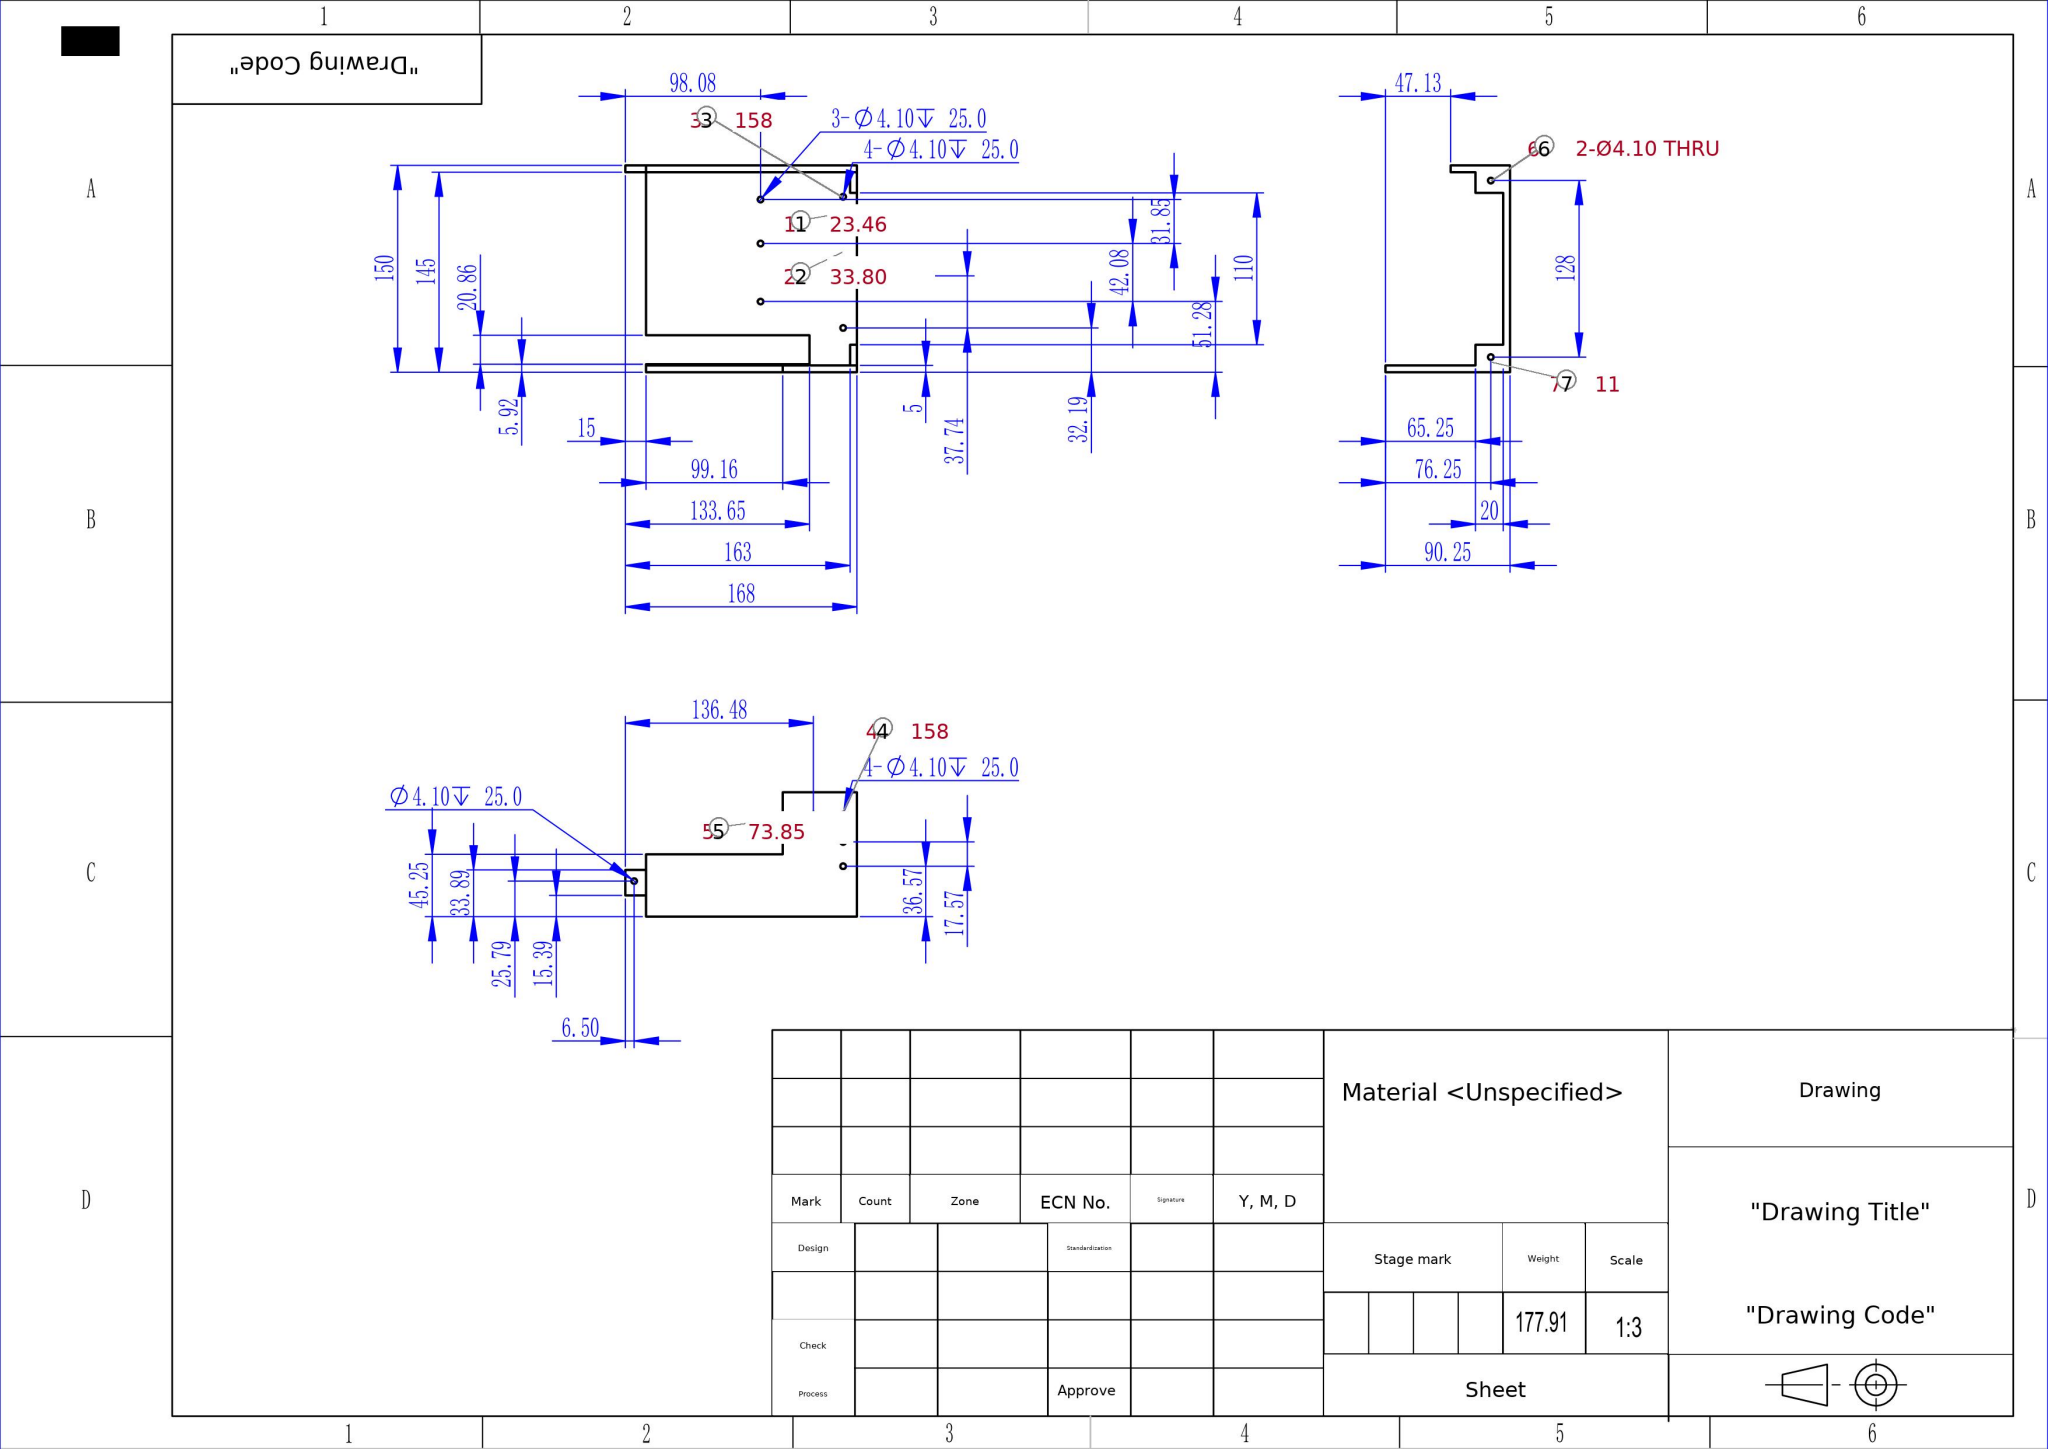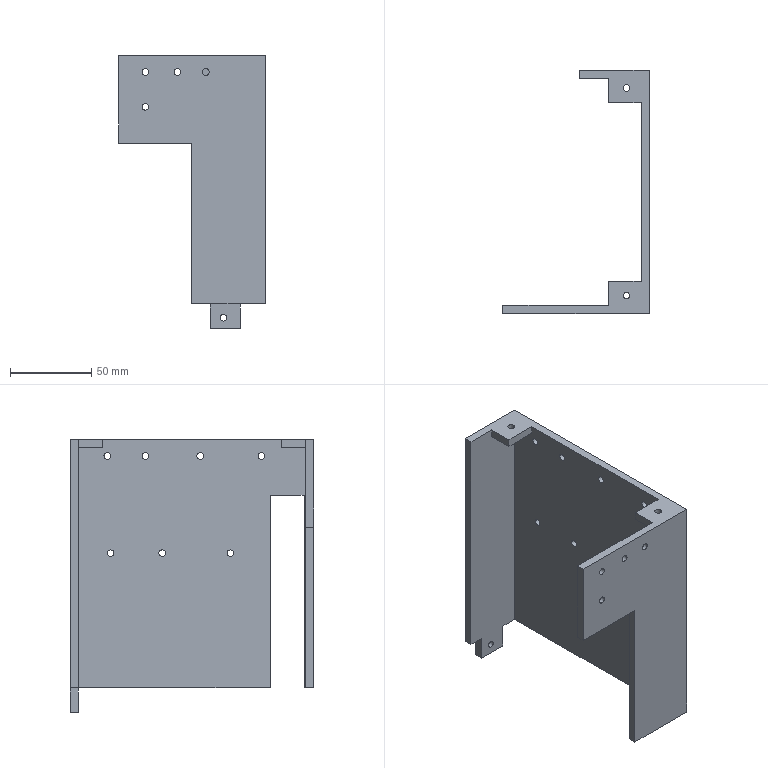Part | SolidWorks | mm | material Unspecified | 1 solid | 54 faces | box 90.25 x 150 x 168 mm | volume 177906 mm3 | cylinder 28 | plane 26 | commonest cylinder face diameters 4.1 x28
build123d program:
from build123d import *

# Parameters (mm, degrees)
BOSS_EXTRUDE1_DEPTH = 153
SKETCH2_W           = 45
SKETCH2_H           = 103.788
CUT_EXTRUDE2_DEPTH  = 104
SKETCH3_W           = 124.99
SKETCH3_H           = 20.86
CUT_EXTRUDE3_DEPTH  = 57
SKETCH4_W           = 20
SKETCH4_H           = 15
SKETCH4_R           = 2.05
BOSS_EXTRUDE2_DEPTH = 5
SKETCH5_W           = 18.5
SKETCH5_H           = 5
BOSS_EXTRUDE3_DEPTH = 15
SKETCH6_R           = 2.05
CUT_EXTRUDE4_DEPTH  = 25
SKETCH7_R           = 2.05
CUT_EXTRUDE5_DEPTH  = 25
SKETCH8_R           = 2.05
CUT_EXTRUDE6_DEPTH  = 25
SKETCH9_R           = 2.05
CUT_EXTRUDE7_DEPTH  = 25


with BuildPart() as part:
    # Sketch1 → Boss-Extrude1 (new body)
    with BuildSketch(Plane.XY):
        Polygon((0, 0), (38.12, 0), (38.12, -140), (-47.13, -140), (-47.13, -145), (43.12, -145), (43.12, 5), (0, 5), align=None)
    extrude(amount=BOSS_EXTRUDE1_DEPTH)

    # Sketch2 → Cut-Extrude2 (cut)
    with BuildSketch(Plane.XZ.offset(145)):
        with Locations((-24.63, 47.262)):
            Rectangle(SKETCH2_W, SKETCH2_H)
    extrude(amount=-CUT_EXTRUDE2_DEPTH, mode=Mode.SUBTRACT)

    # Sketch3 → Cut-Extrude3 (cut)
    with BuildSketch(Plane(origin=(43.12, 0, 0), x_dir=(0, 0, -1), z_dir=(1, 0, 0))):
        with Locations((-56.153, -128.648)):
            Rectangle(SKETCH3_W, SKETCH3_H)
    extrude(amount=-CUT_EXTRUDE3_DEPTH, mode=Mode.SUBTRACT)

    # Sketch4 → Boss-Extrude2 (add)
    # profile 1 of 2: a face of its own
    with BuildSketch(Plane.XY.offset(153)):
        with Locations((28.12, -132.5)):
            Rectangle(SKETCH4_W, SKETCH4_H)
        with Locations((29.12, -134)):
            Circle(SKETCH4_R, mode=Mode.SUBTRACT)
    # profile 2 of 2: a face of its own
    with BuildSketch(Plane.XY.offset(153)):
        with Locations((28.12, -7.5)):
            Rectangle(SKETCH4_W, SKETCH4_H)
        with Locations((29.12, -6)):
            Circle(SKETCH4_R, mode=Mode.SUBTRACT)
    extrude(amount=-BOSS_EXTRUDE2_DEPTH)

    # Sketch5 → Boss-Extrude3 (add)
    with BuildSketch(Plane(origin=(0, 0, 0), x_dir=(-1, 0, 0), z_dir=(0, 0, -1))):
        with Locations((-18.48, 2.5)):
            Rectangle(SKETCH5_W, SKETCH5_H)
    extrude(amount=BOSS_EXTRUDE3_DEPTH)

    # Sketch6 → Cut-Extrude4 (cut)
    with BuildSketch(Plane(origin=(43.12, 0, 0), x_dir=(0, 0, -1), z_dir=(1, 0, 0))):
        with Locations(Location((-143, -112.807, 0), (0, 0, 90))):
            Circle(SKETCH6_R)
        with Locations(Location((-143, -75.069, 0), (0, 0, 90))):
            Circle(SKETCH6_R)
        with Locations(Location((-143, -41.275, 0), (0, 0, 90))):
            Circle(SKETCH6_R)
        with Locations(Location((-143, -17.806, 0), (0, 0, 90))):
            Circle(SKETCH6_R)
    extrude(amount=-CUT_EXTRUDE4_DEPTH, mode=Mode.SUBTRACT)

    # Sketch7 → Cut-Extrude5 (cut)
    with BuildSketch(Plane(origin=(0, 5, 0), x_dir=(1, 0, 0), z_dir=(0, 1, 0))):
        with Locations(Location((17.333, 8.5, 0), (0, 0, 270))):
            Circle(SKETCH7_R)
    extrude(amount=-CUT_EXTRUDE5_DEPTH, mode=Mode.SUBTRACT)

    # Sketch8 → Cut-Extrude6 (cut)
    with BuildSketch(Plane(origin=(43.12, 0, 0), x_dir=(0, 0, -1), z_dir=(1, 0, 0))):
        with Locations(Location((-83.081, -19.794, 0), (0, 0, 90))):
            Circle(SKETCH8_R)
        with Locations(Location((-83.081, -51.644, 0), (0, 0, 90))):
            Circle(SKETCH8_R)
        with Locations(Location((-83.081, -93.72, 0), (0, 0, 90))):
            Circle(SKETCH8_R)
    extrude(amount=-CUT_EXTRUDE6_DEPTH, mode=Mode.SUBTRACT)

    # Sketch9 → Cut-Extrude7 (cut)
    with BuildSketch(Plane.XZ.offset(145)):
        with Locations((-30.73, 143)):
            Circle(SKETCH9_R)
        with Locations((-11.017, 143)):
            Circle(SKETCH9_R)
        with Locations((6.555, 143)):
            Circle(SKETCH9_R)
        with Locations((-30.73, 121.48)):
            Circle(SKETCH9_R)
    extrude(amount=-CUT_EXTRUDE7_DEPTH, mode=Mode.SUBTRACT)


solid = part.part